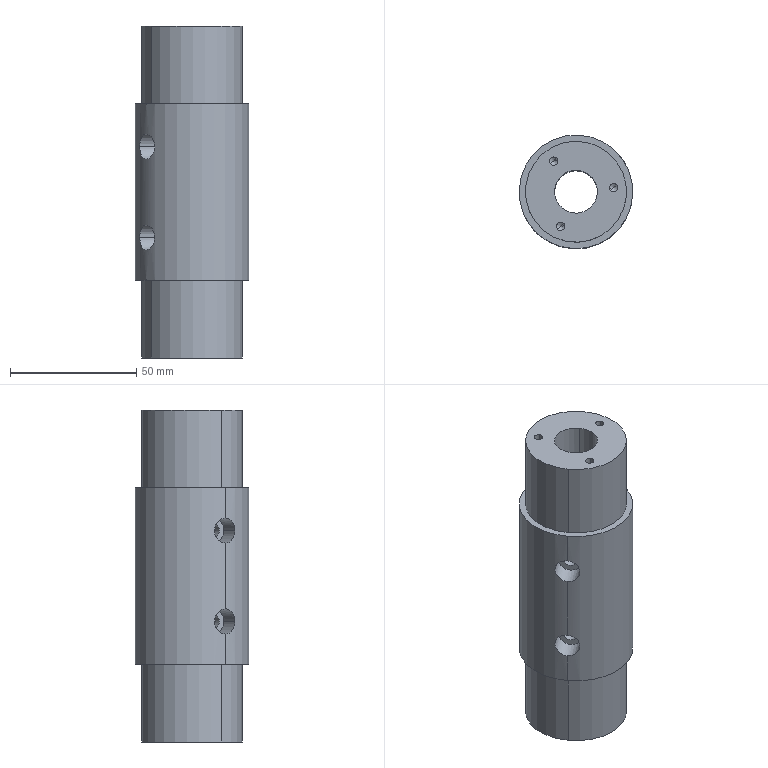Component | SolidWorks | XT-1-14-2-1 | 1 solid | 50 faces | box 45 x 45 x 131.5 mm | volume 156065 mm3 | cylinder 32 | cone 12 | plane 6 | commonest cylinder face diameters 3.3 x12 10 x4 5.5 x4 4.2 x4 40 x4 17 x2 45 x2
build123d program:
from build123d import *

# Parameters (mm, degrees)
SKETCH2_R                                       = 8.5
CUT_EXTRUDE1_DEPTH                              = 136.295
CIRPATTERN1_COUNT                               = 3
CIRPATTERN2_COUNT                               = 3
M5_TAPPED_HOLE1_D                               = 4.2
M5_HEX_SOCKET_HEAD_CAP_SCREW_CBORE1_D           = 5.5
M5_HEX_SOCKET_HEAD_CAP_SCREW_CBORE1_DEPTH       = 20
M5_HEX_SOCKET_HEAD_CAP_SCREW_CBORE1_CBORE_D     = 10
M5_HEX_SOCKET_HEAD_CAP_SCREW_CBORE1_CBORE_DEPTH = 8
M5_HEX_SOCKET_HEAD_CAP_SCREW_CBORE1_TIP         = 1.652


with BuildPart() as part:
    # Sketch1 → Revolve1 (revolve)
    with BuildSketch(Plane.XY, mode=Mode.PRIVATE) as revolve1_sk:
        Polygon((0, 0), (0, -131.5), (20, -131.5), (20, -100.75), (22.5, -100.75), (22.5, -30.75), (20, -30.75), (20, 0), align=None)
    revolve(revolve1_sk.sketch.rotate(Axis((0, 0, 0), (0, -1, 0)), 90), axis=Axis((0, 0, 0), (0, -1, 0)))

    # Sketch2 → Cut-Extrude1 (cut, through all)
    with BuildSketch(Plane.XZ.offset(131.5)):
        with Locations(Location((0, 0, 0), (0, 0, 270))):
            Circle(SKETCH2_R)
    extrude(amount=-CUT_EXTRUDE1_DEPTH, mode=Mode.SUBTRACT)

    # Sketch3 → M4 Tapped Hole1 (revolve, cut)
    with BuildSketch(Plane(origin=(15, -131.5, 0), x_dir=(0, 0, -1), z_dir=(1, 0, 0))):
        Polygon((0, 0), (0, 15.991), (1.65, 15), (1.65, 0), align=None)
    m4_tapped_hole1 = revolve(axis=Axis((15, -137.85, 0), (0, 1, 0)), mode=Mode.SUBTRACT)

    # CirPattern1: M4 Tapped Hole1 ×3 about axis
    cirpattern1_axis = Axis((0, 0, 0), (0, 1, 0))
    for i in range(1, CIRPATTERN1_COUNT):
        add(m4_tapped_hole1.rotate(cirpattern1_axis, i * 360 / CIRPATTERN1_COUNT), mode=Mode.SUBTRACT)

    # Sketch5 → M4 Tapped Hole2 (revolve, cut)
    with BuildSketch(Plane(origin=(-15, 0, 0), x_dir=(0, 0, 1), z_dir=(1, 0, 0))):
        Polygon((0, 0), (0, 15.991), (1.65, 15), (1.65, 0), align=None)
    m4_tapped_hole2 = revolve(axis=Axis((-15, 6.35, 0), (0, -1, 0)), mode=Mode.SUBTRACT)

    # CirPattern2: M4 Tapped Hole2 ×3 about axis
    cirpattern2_axis = Axis((0, 0, 0), (0, 1, 0))
    for i in range(1, CIRPATTERN2_COUNT):
        add(m4_tapped_hole2.rotate(cirpattern2_axis, i * 360 / CIRPATTERN2_COUNT), mode=Mode.SUBTRACT)

    # M5 Tapped Hole1 (through all)
    with Locations(Plane.XY.offset(22.5)):
        with Locations((0, -83.75), (0, -47.75)):
            Hole(M5_TAPPED_HOLE1_D / 2)

    # M5 Hex Socket Head Cap Screw CBORE1
    with Locations(Plane.XY.offset(22.5)):
        with Locations((0, -47.75), (0, -83.75)):
            CounterBoreHole(M5_HEX_SOCKET_HEAD_CAP_SCREW_CBORE1_D / 2, M5_HEX_SOCKET_HEAD_CAP_SCREW_CBORE1_CBORE_D / 2, M5_HEX_SOCKET_HEAD_CAP_SCREW_CBORE1_CBORE_DEPTH, depth=M5_HEX_SOCKET_HEAD_CAP_SCREW_CBORE1_DEPTH)
            with Locations((0, 0, -(M5_HEX_SOCKET_HEAD_CAP_SCREW_CBORE1_DEPTH + M5_HEX_SOCKET_HEAD_CAP_SCREW_CBORE1_TIP / 2))):  # 118° drill point
                Cone(0, M5_HEX_SOCKET_HEAD_CAP_SCREW_CBORE1_D / 2, M5_HEX_SOCKET_HEAD_CAP_SCREW_CBORE1_TIP, mode=Mode.SUBTRACT)


solid = part.part

# Placed as in the assembly
solid = solid.moved(Location((499.783, -234.615, -7), (90, -53.906, 0)))